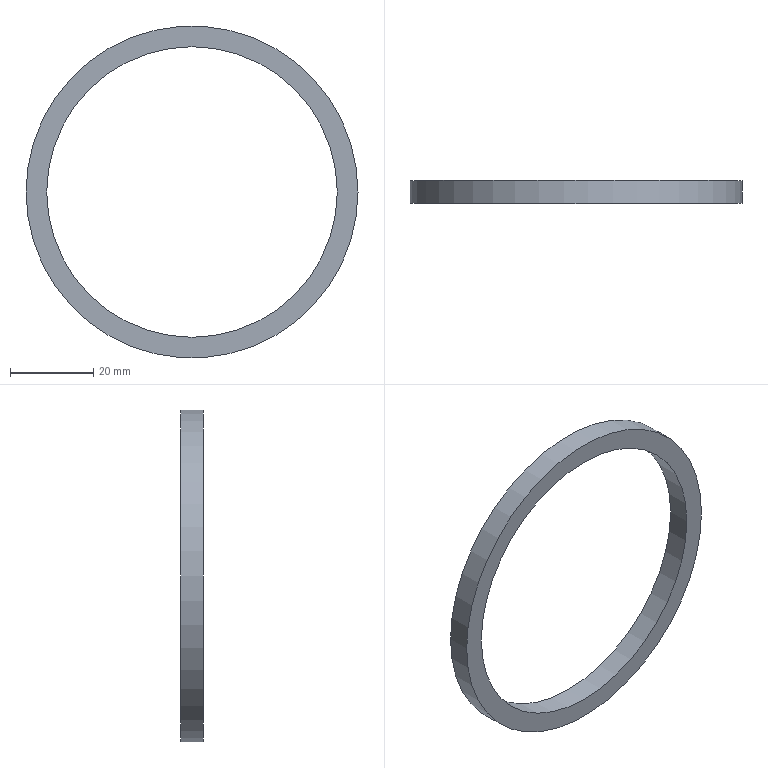Component | NX | ADJUSTING_RING | 1 solid | 4 faces | box 80 x 5.5 x 80 mm | volume 6480 mm3 | cylinder 2 | plane 2 | commonest cylinder face diameters 80 x1 70 x1
STEP:
#1=CARTESIAN_POINT('',(0.,0.,0.));
#2=DIRECTION('',(0.,0.,1.));
#3=DIRECTION('',(1.,0.,0.));
#4=AXIS2_PLACEMENT_3D('',#1,#2,#3);
#5=CARTESIAN_POINT('',(418.803,97.,-135.));
#6=VERTEX_POINT('',#5);
#7=CARTESIAN_POINT('',(378.803,97.,-135.));
#8=DIRECTION('',(0.,-1.,0.));
#9=DIRECTION('',(1.,0.,0.));
#10=AXIS2_PLACEMENT_3D('',#7,#8,#9);
#11=CIRCLE('',#10,40.);
#12=CARTESIAN_POINT('',(378.803,97.,-135.));
#13=DIRECTION('',(0.,1.,0.));
#14=DIRECTION('',(0.,0.,1.));
#15=AXIS2_PLACEMENT_3D('',#12,#13,#14);
#16=CYLINDRICAL_SURFACE('',#15,40.);
#17=CARTESIAN_POINT('',(7.854,0.));
#18=DIRECTION('',(-1.,0.));
#19=VECTOR('',#18,1.);
#20=LINE('',#17,#19);
#21=(GEOMETRIC_REPRESENTATION_CONTEXT(2)PARAMETRIC_REPRESENTATION_CONTEXT()REPRESENTATION_CONTEXT('',''));
#22=DEFINITIONAL_REPRESENTATION('',(#20),#21);
#23=PCURVE('',#16,#22);
#24=CARTESIAN_POINT('',(378.803,97.,-135.));
#25=DIRECTION('',(0.,-1.,0.));
#26=DIRECTION('',(0.,0.,-1.));
#27=AXIS2_PLACEMENT_3D('',#24,#25,#26);
#28=PLANE('',#27);
#29=CARTESIAN_POINT('',(0.,0.));
#30=DIRECTION('',(0.,1.));
#31=AXIS2_PLACEMENT_2D('',#29,#30);
#32=CIRCLE('',#31,40.);
#33=(GEOMETRIC_REPRESENTATION_CONTEXT(2)PARAMETRIC_REPRESENTATION_CONTEXT()REPRESENTATION_CONTEXT('',''));
#34=DEFINITIONAL_REPRESENTATION('',(#32),#33);
#35=PCURVE('',#28,#34);
#36=SURFACE_CURVE('',#11,(#23,#35),.PCURVE_S1.);
#37=EDGE_CURVE('',#6,#6,#36,.T.);
#38=ORIENTED_EDGE('',*,*,#37,.F.);
#39=CARTESIAN_POINT('',(418.803,102.5,-135.));
#40=VERTEX_POINT('',#39);
#41=CARTESIAN_POINT('',(418.803,97.,-135.));
#42=CARTESIAN_POINT('',(418.803,102.5,-135.));
#43=B_SPLINE_CURVE_WITH_KNOTS('',1,(#41,#42),.UNSPECIFIED.,.F.,.F.,(2,2),(0.,5.5),.PIECEWISE_BEZIER_KNOTS.);
#44=CARTESIAN_POINT('',(7.854,0.));
#45=DIRECTION('',(0.,1.));
#46=VECTOR('',#45,1.);
#47=LINE('',#44,#46);
#48=(GEOMETRIC_REPRESENTATION_CONTEXT(2)PARAMETRIC_REPRESENTATION_CONTEXT()REPRESENTATION_CONTEXT('',''));
#49=DEFINITIONAL_REPRESENTATION('',(#47),#48);
#50=PCURVE('',#16,#49);
#51=CARTESIAN_POINT('',(1.571,0.));
#52=DIRECTION('',(0.,1.));
#53=VECTOR('',#52,1.);
#54=LINE('',#51,#53);
#55=(GEOMETRIC_REPRESENTATION_CONTEXT(2)PARAMETRIC_REPRESENTATION_CONTEXT()REPRESENTATION_CONTEXT('',''));
#56=DEFINITIONAL_REPRESENTATION('',(#54),#55);
#57=PCURVE('',#16,#56);
#58=SEAM_CURVE('',#43,(#50,#57),.PCURVE_S1.);
#59=EDGE_CURVE('',#6,#40,#58,.T.);
#60=ORIENTED_EDGE('',*,*,#59,.T.);
#61=CARTESIAN_POINT('',(378.803,102.5,-135.));
#62=DIRECTION('',(0.,-1.,0.));
#63=DIRECTION('',(1.,0.,0.));
#64=AXIS2_PLACEMENT_3D('',#61,#62,#63);
#65=CIRCLE('',#64,40.);
#66=CARTESIAN_POINT('',(7.854,5.5));
#67=DIRECTION('',(-1.,0.));
#68=VECTOR('',#67,1.);
#69=LINE('',#66,#68);
#70=(GEOMETRIC_REPRESENTATION_CONTEXT(2)PARAMETRIC_REPRESENTATION_CONTEXT()REPRESENTATION_CONTEXT('',''));
#71=DEFINITIONAL_REPRESENTATION('',(#69),#70);
#72=PCURVE('',#16,#71);
#73=CARTESIAN_POINT('',(378.803,102.5,-135.));
#74=DIRECTION('',(0.,-1.,0.));
#75=DIRECTION('',(0.,0.,-1.));
#76=AXIS2_PLACEMENT_3D('',#73,#74,#75);
#77=PLANE('',#76);
#78=CARTESIAN_POINT('',(0.,0.));
#79=DIRECTION('',(0.,1.));
#80=AXIS2_PLACEMENT_2D('',#78,#79);
#81=CIRCLE('',#80,40.);
#82=(GEOMETRIC_REPRESENTATION_CONTEXT(2)PARAMETRIC_REPRESENTATION_CONTEXT()REPRESENTATION_CONTEXT('',''));
#83=DEFINITIONAL_REPRESENTATION('',(#81),#82);
#84=PCURVE('',#77,#83);
#85=SURFACE_CURVE('',#65,(#72,#84),.PCURVE_S1.);
#86=EDGE_CURVE('',#40,#40,#85,.T.);
#87=ORIENTED_EDGE('',*,*,#86,.T.);
#88=ORIENTED_EDGE('',*,*,#59,.F.);
#89=EDGE_LOOP('',(#38,#60,#87,#88));
#90=FACE_BOUND('',#89,.T.);
#91=ADVANCED_FACE('',(#90),#16,.T.);
#92=CARTESIAN_POINT('',(413.803,97.,-135.));
#93=VERTEX_POINT('',#92);
#94=CARTESIAN_POINT('',(378.803,97.,-135.));
#95=DIRECTION('',(0.,-1.,0.));
#96=DIRECTION('',(1.,0.,0.));
#97=AXIS2_PLACEMENT_3D('',#94,#95,#96);
#98=CIRCLE('',#97,35.);
#99=CARTESIAN_POINT('',(378.803,97.,-135.));
#100=DIRECTION('',(0.,1.,0.));
#101=DIRECTION('',(0.,0.,1.));
#102=AXIS2_PLACEMENT_3D('',#99,#100,#101);
#103=CYLINDRICAL_SURFACE('',#102,35.);
#104=CARTESIAN_POINT('',(7.854,0.));
#105=DIRECTION('',(-1.,0.));
#106=VECTOR('',#105,1.);
#107=LINE('',#104,#106);
#108=(GEOMETRIC_REPRESENTATION_CONTEXT(2)PARAMETRIC_REPRESENTATION_CONTEXT()REPRESENTATION_CONTEXT('',''));
#109=DEFINITIONAL_REPRESENTATION('',(#107),#108);
#110=PCURVE('',#103,#109);
#111=CARTESIAN_POINT('',(0.,0.));
#112=DIRECTION('',(0.,1.));
#113=AXIS2_PLACEMENT_2D('',#111,#112);
#114=CIRCLE('',#113,35.);
#115=(GEOMETRIC_REPRESENTATION_CONTEXT(2)PARAMETRIC_REPRESENTATION_CONTEXT()REPRESENTATION_CONTEXT('',''));
#116=DEFINITIONAL_REPRESENTATION('',(#114),#115);
#117=PCURVE('',#28,#116);
#118=SURFACE_CURVE('',#98,(#110,#117),.PCURVE_S1.);
#119=EDGE_CURVE('',#93,#93,#118,.T.);
#120=ORIENTED_EDGE('',*,*,#119,.F.);
#121=CARTESIAN_POINT('',(413.803,102.5,-135.));
#122=VERTEX_POINT('',#121);
#123=CARTESIAN_POINT('',(413.803,97.,-135.));
#124=CARTESIAN_POINT('',(413.803,102.5,-135.));
#125=B_SPLINE_CURVE_WITH_KNOTS('',1,(#123,#124),.UNSPECIFIED.,.F.,.F.,(2,2),(0.,5.5),.PIECEWISE_BEZIER_KNOTS.);
#126=CARTESIAN_POINT('',(7.854,0.));
#127=DIRECTION('',(0.,1.));
#128=VECTOR('',#127,1.);
#129=LINE('',#126,#128);
#130=(GEOMETRIC_REPRESENTATION_CONTEXT(2)PARAMETRIC_REPRESENTATION_CONTEXT()REPRESENTATION_CONTEXT('',''));
#131=DEFINITIONAL_REPRESENTATION('',(#129),#130);
#132=PCURVE('',#103,#131);
#133=CARTESIAN_POINT('',(1.571,0.));
#134=DIRECTION('',(0.,1.));
#135=VECTOR('',#134,1.);
#136=LINE('',#133,#135);
#137=(GEOMETRIC_REPRESENTATION_CONTEXT(2)PARAMETRIC_REPRESENTATION_CONTEXT()REPRESENTATION_CONTEXT('',''));
#138=DEFINITIONAL_REPRESENTATION('',(#136),#137);
#139=PCURVE('',#103,#138);
#140=SEAM_CURVE('',#125,(#132,#139),.PCURVE_S1.);
#141=EDGE_CURVE('',#93,#122,#140,.T.);
#142=ORIENTED_EDGE('',*,*,#141,.T.);
#143=CARTESIAN_POINT('',(378.803,102.5,-135.));
#144=DIRECTION('',(0.,-1.,0.));
#145=DIRECTION('',(1.,0.,0.));
#146=AXIS2_PLACEMENT_3D('',#143,#144,#145);
#147=CIRCLE('',#146,35.);
#148=CARTESIAN_POINT('',(7.854,5.5));
#149=DIRECTION('',(-1.,0.));
#150=VECTOR('',#149,1.);
#151=LINE('',#148,#150);
#152=(GEOMETRIC_REPRESENTATION_CONTEXT(2)PARAMETRIC_REPRESENTATION_CONTEXT()REPRESENTATION_CONTEXT('',''));
#153=DEFINITIONAL_REPRESENTATION('',(#151),#152);
#154=PCURVE('',#103,#153);
#155=CARTESIAN_POINT('',(0.,0.));
#156=DIRECTION('',(0.,1.));
#157=AXIS2_PLACEMENT_2D('',#155,#156);
#158=CIRCLE('',#157,35.);
#159=(GEOMETRIC_REPRESENTATION_CONTEXT(2)PARAMETRIC_REPRESENTATION_CONTEXT()REPRESENTATION_CONTEXT('',''));
#160=DEFINITIONAL_REPRESENTATION('',(#158),#159);
#161=PCURVE('',#77,#160);
#162=SURFACE_CURVE('',#147,(#154,#161),.PCURVE_S1.);
#163=EDGE_CURVE('',#122,#122,#162,.T.);
#164=ORIENTED_EDGE('',*,*,#163,.T.);
#165=ORIENTED_EDGE('',*,*,#141,.F.);
#166=EDGE_LOOP('',(#120,#142,#164,#165));
#167=FACE_BOUND('',#166,.F.);
#168=ADVANCED_FACE('',(#167),#103,.F.);
#169=ORIENTED_EDGE('',*,*,#37,.T.);
#170=EDGE_LOOP('',(#169));
#171=FACE_BOUND('',#170,.T.);
#172=ORIENTED_EDGE('',*,*,#119,.F.);
#173=EDGE_LOOP('',(#172));
#174=FACE_BOUND('',#173,.T.);
#175=ADVANCED_FACE('',(#171,#174),#28,.T.);
#176=ORIENTED_EDGE('',*,*,#86,.F.);
#177=EDGE_LOOP('',(#176));
#178=FACE_BOUND('',#177,.T.);
#179=ORIENTED_EDGE('',*,*,#163,.T.);
#180=EDGE_LOOP('',(#179));
#181=FACE_BOUND('',#180,.T.);
#182=ADVANCED_FACE('',(#178,#181),#77,.F.);
#183=CLOSED_SHELL('',(#91,#168,#175,#182));
#184=MANIFOLD_SOLID_BREP('',#183);
#185=(LENGTH_UNIT()NAMED_UNIT(*)SI_UNIT(.MILLI.,.METRE.));
#186=UNCERTAINTY_MEASURE_WITH_UNIT(LENGTH_MEASURE(0.00001),#185,'','');
#187=(NAMED_UNIT(*)PLANE_ANGLE_UNIT()SI_UNIT($,.RADIAN.));
#188=(NAMED_UNIT(*)SI_UNIT($,.STERADIAN.)SOLID_ANGLE_UNIT());
#189=(GEOMETRIC_REPRESENTATION_CONTEXT(3)GLOBAL_UNCERTAINTY_ASSIGNED_CONTEXT((#186))GLOBAL_UNIT_ASSIGNED_CONTEXT((#185,#187,#188))REPRESENTATION_CONTEXT('',''));
#190=ADVANCED_BREP_SHAPE_REPRESENTATION('',(#4,#184),#189);